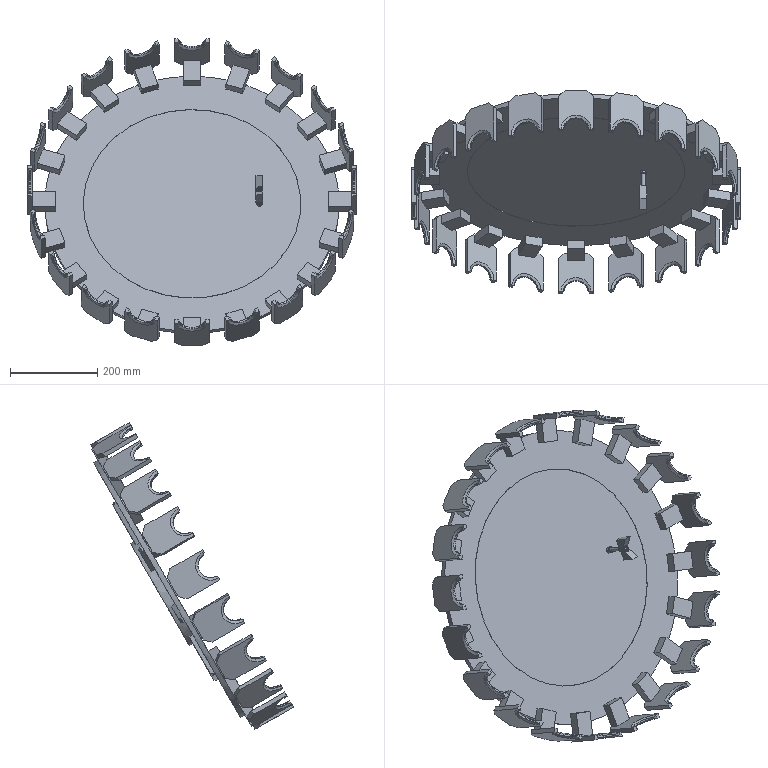Component | NX | SIM15_MAGAZIN | 1 solid | 670 faces | volume 7009512 mm3 | plane 495 | cone 90 | cylinder 83 | torus 2 | commonest cylinder face diameters 55.4 x40 54 x20 495 x8 8 x3 4 x2 270 x1 676 x1 250 x1